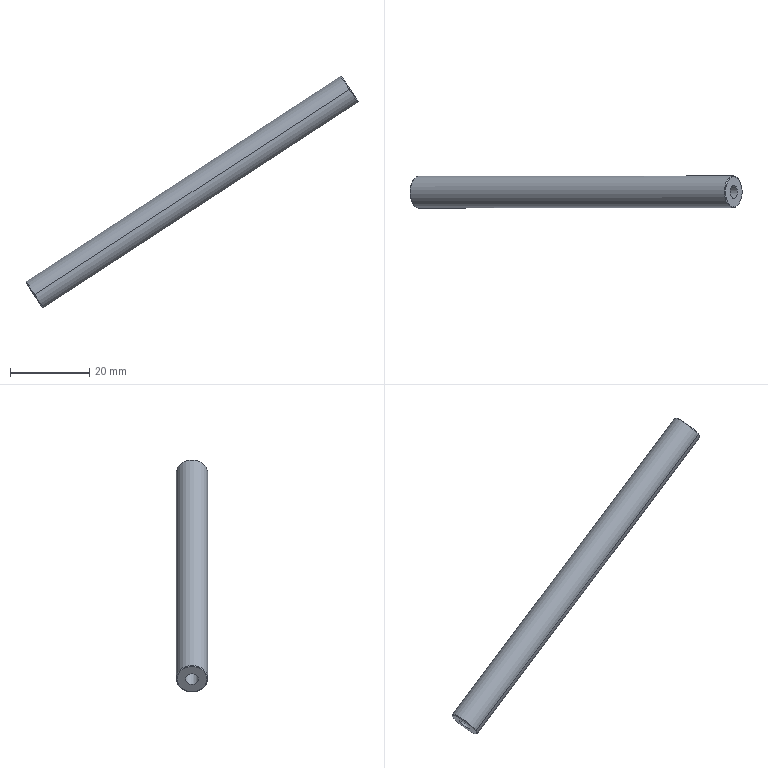Component | SolidWorks | NewSuctionCupGroup-1_GuideRod01-2 | 1 solid | 16 faces | box 83.68 x 8 x 58.45 mm | volume 4596 mm3 | cone 8 | cylinder 6 | plane 2 | commonest cylinder face diameters 3.3 x4 8 x2
build123d program:
from build123d import *

# Parameters (mm, degrees)
SKETCH1_R             = 4
BOSS_EXTRUDE1_DEPTH   = 95
CHAMFER1_SIZE         = 0.2
M4_TAPPED_HOLE1_D     = 3.3
M4_TAPPED_HOLE1_DEPTH = 10.1
M4_TAPPED_HOLE1_TIP   = 0.9914
M4_TAPPED_HOLE2_D     = 3.3
M4_TAPPED_HOLE2_DEPTH = 10.1
M4_TAPPED_HOLE2_TIP   = 0.9914


with BuildPart() as part:
    # Sketch1 → Boss-Extrude1 (new body)
    with BuildSketch(Plane.XY):
        Circle(SKETCH1_R)
    extrude(amount=BOSS_EXTRUDE1_DEPTH)

    # Chamfer1
    chamfer1_edges = [part.edges().sort_by_distance(p)[0] for p in [
        (-4, 0, 0),
        (-4, 0, 95),
    ]]
    chamfer(chamfer1_edges, length=CHAMFER1_SIZE)

    # M4 Tapped Hole1
    with Locations(Plane.XY.offset(95)):
        with Locations((0, 0)):
            Hole(M4_TAPPED_HOLE1_D / 2, depth=M4_TAPPED_HOLE1_DEPTH)
            with Locations((0, 0, -(M4_TAPPED_HOLE1_DEPTH + M4_TAPPED_HOLE1_TIP / 2))):  # 118° drill point
                Cone(0, M4_TAPPED_HOLE1_D / 2, M4_TAPPED_HOLE1_TIP, mode=Mode.SUBTRACT)

    # M4 Tapped Hole2
    with Locations(Plane(origin=(0, 0, 0), x_dir=(-1, 0, 0), z_dir=(0, 0, -1))):
        with Locations((0, 0)):
            Hole(M4_TAPPED_HOLE2_D / 2, depth=M4_TAPPED_HOLE2_DEPTH)
            with Locations((0, 0, -(M4_TAPPED_HOLE2_DEPTH + M4_TAPPED_HOLE2_TIP / 2))):  # 118° drill point
                Cone(0, M4_TAPPED_HOLE2_D / 2, M4_TAPPED_HOLE2_TIP, mode=Mode.SUBTRACT)


solid = part.part

# Placed as in the assembly
solid = solid.moved(Location((-73.051, -140.454, -18.564), (0, 56.835, 67.886)))
STEP:
#1=CARTESIAN_POINT('',(-0.07801,-5.595,1.098));
#2=VERTEX_POINT('',#1);
#3=CARTESIAN_POINT('',(-0.07801,-5.465,1.098));
#4=VERTEX_POINT('',#3);
#5=CARTESIAN_POINT('',(-0.07801,-5.53,1.098));
#6=DIRECTION('',(0.8371,-0.,0.5471));
#7=DIRECTION('',(0.,1.,0.));
#8=AXIS2_PLACEMENT_3D('',#5,#6,#7);
#9=CIRCLE('',#8,0.06496);
#10=EDGE_CURVE('',#2,#4,#9,.T.);
#11=ORIENTED_EDGE('',*,*,#10,.F.);
#12=CARTESIAN_POINT('',(0.2548,-5.595,1.315));
#13=VERTEX_POINT('',#12);
#14=CARTESIAN_POINT('',(0.2548,-5.595,1.315));
#15=DIRECTION('',(0.8371,-0.,0.5471));
#16=VECTOR('',#15,39.37);
#17=LINE('',#14,#16);
#18=EDGE_CURVE('',#2,#13,#17,.T.);
#19=ORIENTED_EDGE('',*,*,#18,.T.);
#20=CARTESIAN_POINT('',(0.2548,-5.465,1.315));
#21=VERTEX_POINT('',#20);
#22=CARTESIAN_POINT('',(0.2548,-5.53,1.315));
#23=DIRECTION('',(0.8371,-0.,0.5471));
#24=DIRECTION('',(0.,1.,0.));
#25=AXIS2_PLACEMENT_3D('',#22,#23,#24);
#26=CIRCLE('',#25,0.06496);
#27=EDGE_CURVE('',#13,#21,#26,.T.);
#28=ORIENTED_EDGE('',*,*,#27,.T.);
#29=CARTESIAN_POINT('',(0.2548,-5.465,1.315));
#30=DIRECTION('',(0.8371,-0.,0.5471));
#31=VECTOR('',#30,39.37);
#32=LINE('',#29,#31);
#33=EDGE_CURVE('',#4,#21,#32,.T.);
#34=ORIENTED_EDGE('',*,*,#33,.F.);
#35=EDGE_LOOP('',(#11,#19,#28,#34));
#36=FACE_OUTER_BOUND('',#35,.T.);
#37=CARTESIAN_POINT('',(0.2548,-5.53,1.315));
#38=DIRECTION('',(0.8371,-0.,0.5471));
#39=DIRECTION('',(0.,1.,0.));
#40=AXIS2_PLACEMENT_3D('',#37,#38,#39);
#41=CYLINDRICAL_SURFACE('',#40,0.06496);
#42=ADVANCED_FACE('',(#36),#41,.F.);
#43=CARTESIAN_POINT('',(-0.1107,-5.53,1.076));
#44=VERTEX_POINT('',#43);
#45=CARTESIAN_POINT('',(-0.07801,-5.465,1.098));
#46=DIRECTION('',(0.4311,0.8572,0.2818));
#47=VECTOR('',#46,39.37);
#48=LINE('',#45,#47);
#49=EDGE_CURVE('',#44,#4,#48,.T.);
#50=ORIENTED_EDGE('',*,*,#49,.F.);
#51=CARTESIAN_POINT('',(-0.07801,-5.595,1.098));
#52=DIRECTION('',(0.4311,-0.8572,0.2818));
#53=VECTOR('',#52,39.37);
#54=LINE('',#51,#53);
#55=EDGE_CURVE('',#44,#2,#54,.T.);
#56=ORIENTED_EDGE('',*,*,#55,.T.);
#57=ORIENTED_EDGE('',*,*,#10,.T.);
#58=EDGE_LOOP('',(#50,#56,#57));
#59=FACE_OUTER_BOUND('',#58,.T.);
#60=CARTESIAN_POINT('',(-0.07801,-5.53,1.098));
#61=DIRECTION('',(0.8371,-0.,0.5471));
#62=DIRECTION('',(0.,1.,0.));
#63=AXIS2_PLACEMENT_3D('',#60,#61,#62);
#64=CONICAL_SURFACE('',#63,0.06496,1.03);
#65=ADVANCED_FACE('',(#59),#64,.F.);
#66=CARTESIAN_POINT('',(-2.543,-5.465,-0.5133));
#67=VERTEX_POINT('',#66);
#68=CARTESIAN_POINT('',(-2.543,-5.595,-0.5133));
#69=VERTEX_POINT('',#68);
#70=CARTESIAN_POINT('',(-2.543,-5.53,-0.5133));
#71=DIRECTION('',(-0.8371,0.,-0.5471));
#72=DIRECTION('',(0.,-1.,0.));
#73=AXIS2_PLACEMENT_3D('',#70,#71,#72);
#74=CIRCLE('',#73,0.06496);
#75=EDGE_CURVE('',#67,#69,#74,.T.);
#76=ORIENTED_EDGE('',*,*,#75,.F.);
#77=CARTESIAN_POINT('',(-2.876,-5.465,-0.7309));
#78=VERTEX_POINT('',#77);
#79=CARTESIAN_POINT('',(-2.876,-5.465,-0.7309));
#80=DIRECTION('',(-0.8371,0.,-0.5471));
#81=VECTOR('',#80,39.37);
#82=LINE('',#79,#81);
#83=EDGE_CURVE('',#67,#78,#82,.T.);
#84=ORIENTED_EDGE('',*,*,#83,.T.);
#85=CARTESIAN_POINT('',(-2.876,-5.595,-0.7309));
#86=VERTEX_POINT('',#85);
#87=CARTESIAN_POINT('',(-2.876,-5.53,-0.7309));
#88=DIRECTION('',(-0.8371,0.,-0.5471));
#89=DIRECTION('',(0.,-1.,0.));
#90=AXIS2_PLACEMENT_3D('',#87,#88,#89);
#91=CIRCLE('',#90,0.06496);
#92=EDGE_CURVE('',#78,#86,#91,.T.);
#93=ORIENTED_EDGE('',*,*,#92,.T.);
#94=CARTESIAN_POINT('',(-2.876,-5.595,-0.7309));
#95=DIRECTION('',(-0.8371,0.,-0.5471));
#96=VECTOR('',#95,39.37);
#97=LINE('',#94,#96);
#98=EDGE_CURVE('',#69,#86,#97,.T.);
#99=ORIENTED_EDGE('',*,*,#98,.F.);
#100=EDGE_LOOP('',(#76,#84,#93,#99));
#101=FACE_OUTER_BOUND('',#100,.T.);
#102=CARTESIAN_POINT('',(-2.876,-5.53,-0.7309));
#103=DIRECTION('',(-0.8371,0.,-0.5471));
#104=DIRECTION('',(0.,-1.,0.));
#105=AXIS2_PLACEMENT_3D('',#102,#103,#104);
#106=CYLINDRICAL_SURFACE('',#105,0.06496);
#107=ADVANCED_FACE('',(#101),#106,.F.);
#108=CARTESIAN_POINT('',(-2.51,-5.53,-0.492));
#109=VERTEX_POINT('',#108);
#110=CARTESIAN_POINT('',(-2.543,-5.595,-0.5133));
#111=DIRECTION('',(-0.4311,-0.8572,-0.2818));
#112=VECTOR('',#111,39.37);
#113=LINE('',#110,#112);
#114=EDGE_CURVE('',#109,#69,#113,.T.);
#115=ORIENTED_EDGE('',*,*,#114,.F.);
#116=CARTESIAN_POINT('',(-2.543,-5.465,-0.5133));
#117=DIRECTION('',(-0.4311,0.8572,-0.2818));
#118=VECTOR('',#117,39.37);
#119=LINE('',#116,#118);
#120=EDGE_CURVE('',#109,#67,#119,.T.);
#121=ORIENTED_EDGE('',*,*,#120,.T.);
#122=ORIENTED_EDGE('',*,*,#75,.T.);
#123=EDGE_LOOP('',(#115,#121,#122));
#124=FACE_OUTER_BOUND('',#123,.T.);
#125=CARTESIAN_POINT('',(-2.543,-5.53,-0.5133));
#126=DIRECTION('',(-0.8371,0.,-0.5471));
#127=DIRECTION('',(0.,-1.,0.));
#128=AXIS2_PLACEMENT_3D('',#125,#126,#127);
#129=CONICAL_SURFACE('',#128,0.06496,1.03);
#130=ADVANCED_FACE('',(#124),#129,.F.);
#131=CARTESIAN_POINT('',(-2.876,-5.679,-0.7309));
#132=VERTEX_POINT('',#131);
#133=CARTESIAN_POINT('',(-2.876,-5.38,-0.7309));
#134=VERTEX_POINT('',#133);
#135=CARTESIAN_POINT('',(-2.876,-5.53,-0.7309));
#136=DIRECTION('',(-0.8371,0.,-0.5471));
#137=DIRECTION('',(0.,-1.,0.));
#138=AXIS2_PLACEMENT_3D('',#135,#136,#137);
#139=CIRCLE('',#138,0.1496);
#140=EDGE_CURVE('',#132,#134,#139,.T.);
#141=ORIENTED_EDGE('',*,*,#140,.F.);
#142=CARTESIAN_POINT('',(-2.869,-5.687,-0.7266));
#143=VERTEX_POINT('',#142);
#144=CARTESIAN_POINT('',(-2.876,-5.679,-0.7309));
#145=DIRECTION('',(0.5919,-0.7071,0.3868));
#146=VECTOR('',#145,39.37);
#147=LINE('',#144,#146);
#148=EDGE_CURVE('',#132,#143,#147,.T.);
#149=ORIENTED_EDGE('',*,*,#148,.T.);
#150=CARTESIAN_POINT('',(-2.869,-5.372,-0.7266));
#151=VERTEX_POINT('',#150);
#152=CARTESIAN_POINT('',(-2.869,-5.53,-0.7266));
#153=DIRECTION('',(0.8371,-0.,0.5471));
#154=DIRECTION('',(0.,-1.,-0.));
#155=AXIS2_PLACEMENT_3D('',#152,#153,#154);
#156=CIRCLE('',#155,0.1575);
#157=EDGE_CURVE('',#151,#143,#156,.T.);
#158=ORIENTED_EDGE('',*,*,#157,.F.);
#159=CARTESIAN_POINT('',(-2.876,-5.38,-0.7309));
#160=DIRECTION('',(0.5919,0.7071,0.3868));
#161=VECTOR('',#160,39.37);
#162=LINE('',#159,#161);
#163=EDGE_CURVE('',#134,#151,#162,.T.);
#164=ORIENTED_EDGE('',*,*,#163,.F.);
#165=EDGE_LOOP('',(#141,#149,#158,#164));
#166=FACE_OUTER_BOUND('',#165,.T.);
#167=CARTESIAN_POINT('',(-2.876,-5.53,-0.7309));
#168=DIRECTION('',(0.8371,-0.,0.5471));
#169=DIRECTION('',(0.,1.,-0.));
#170=AXIS2_PLACEMENT_3D('',#167,#168,#169);
#171=CONICAL_SURFACE('',#170,0.1496,0.7854);
#172=ADVANCED_FACE('',(#166),#171,.T.);
#173=CARTESIAN_POINT('',(0.2548,-5.38,1.315));
#174=VERTEX_POINT('',#173);
#175=CARTESIAN_POINT('',(0.2548,-5.679,1.315));
#176=VERTEX_POINT('',#175);
#177=CARTESIAN_POINT('',(0.2548,-5.53,1.315));
#178=DIRECTION('',(0.8371,-0.,0.5471));
#179=DIRECTION('',(-0.,-1.,0.));
#180=AXIS2_PLACEMENT_3D('',#177,#178,#179);
#181=CIRCLE('',#180,0.1496);
#182=EDGE_CURVE('',#174,#176,#181,.T.);
#183=ORIENTED_EDGE('',*,*,#182,.F.);
#184=CARTESIAN_POINT('',(0.2483,-5.372,1.311));
#185=VERTEX_POINT('',#184);
#186=CARTESIAN_POINT('',(0.2483,-5.372,1.311));
#187=DIRECTION('',(-0.5919,0.7071,-0.3868));
#188=VECTOR('',#187,39.37);
#189=LINE('',#186,#188);
#190=EDGE_CURVE('',#174,#185,#189,.T.);
#191=ORIENTED_EDGE('',*,*,#190,.T.);
#192=CARTESIAN_POINT('',(0.2483,-5.687,1.311));
#193=VERTEX_POINT('',#192);
#194=CARTESIAN_POINT('',(0.2483,-5.53,1.311));
#195=DIRECTION('',(-0.8371,0.,-0.5471));
#196=DIRECTION('',(-0.,-1.,0.));
#197=AXIS2_PLACEMENT_3D('',#194,#195,#196);
#198=CIRCLE('',#197,0.1575);
#199=EDGE_CURVE('',#193,#185,#198,.T.);
#200=ORIENTED_EDGE('',*,*,#199,.F.);
#201=CARTESIAN_POINT('',(0.2483,-5.687,1.311));
#202=DIRECTION('',(-0.5919,-0.7071,-0.3868));
#203=VECTOR('',#202,39.37);
#204=LINE('',#201,#203);
#205=EDGE_CURVE('',#176,#193,#204,.T.);
#206=ORIENTED_EDGE('',*,*,#205,.F.);
#207=EDGE_LOOP('',(#183,#191,#200,#206));
#208=FACE_OUTER_BOUND('',#207,.T.);
#209=CARTESIAN_POINT('',(0.2483,-5.53,1.311));
#210=DIRECTION('',(-0.8371,0.,-0.5471));
#211=DIRECTION('',(-0.,-1.,0.));
#212=AXIS2_PLACEMENT_3D('',#209,#210,#211);
#213=CONICAL_SURFACE('',#212,0.1575,0.7854);
#214=ADVANCED_FACE('',(#208),#213,.T.);
#215=ORIENTED_EDGE('',*,*,#157,.T.);
#216=CARTESIAN_POINT('',(-2.876,-5.687,-0.7309));
#217=DIRECTION('',(0.8371,-0.,0.5471));
#218=VECTOR('',#217,39.37);
#219=LINE('',#216,#218);
#220=EDGE_CURVE('',#143,#193,#219,.T.);
#221=ORIENTED_EDGE('',*,*,#220,.T.);
#222=ORIENTED_EDGE('',*,*,#199,.T.);
#223=CARTESIAN_POINT('',(-2.876,-5.372,-0.7309));
#224=DIRECTION('',(0.8371,-0.,0.5471));
#225=VECTOR('',#224,39.37);
#226=LINE('',#223,#225);
#227=EDGE_CURVE('',#151,#185,#226,.T.);
#228=ORIENTED_EDGE('',*,*,#227,.F.);
#229=EDGE_LOOP('',(#215,#221,#222,#228));
#230=FACE_OUTER_BOUND('',#229,.T.);
#231=CARTESIAN_POINT('',(-2.876,-5.53,-0.7309));
#232=DIRECTION('',(0.8371,-0.,0.5471));
#233=DIRECTION('',(0.,1.,-0.));
#234=AXIS2_PLACEMENT_3D('',#231,#232,#233);
#235=CYLINDRICAL_SURFACE('',#234,0.1575);
#236=ADVANCED_FACE('',(#230),#235,.T.);
#237=ORIENTED_EDGE('',*,*,#220,.F.);
#238=CARTESIAN_POINT('',(-2.869,-5.53,-0.7266));
#239=DIRECTION('',(0.8371,-0.,0.5471));
#240=DIRECTION('',(-0.,-1.,0.));
#241=AXIS2_PLACEMENT_3D('',#238,#239,#240);
#242=CIRCLE('',#241,0.1575);
#243=EDGE_CURVE('',#143,#151,#242,.T.);
#244=ORIENTED_EDGE('',*,*,#243,.T.);
#245=ORIENTED_EDGE('',*,*,#227,.T.);
#246=CARTESIAN_POINT('',(0.2483,-5.53,1.311));
#247=DIRECTION('',(-0.8371,0.,-0.5471));
#248=DIRECTION('',(-0.,-1.,0.));
#249=AXIS2_PLACEMENT_3D('',#246,#247,#248);
#250=CIRCLE('',#249,0.1575);
#251=EDGE_CURVE('',#185,#193,#250,.T.);
#252=ORIENTED_EDGE('',*,*,#251,.T.);
#253=EDGE_LOOP('',(#237,#244,#245,#252));
#254=FACE_OUTER_BOUND('',#253,.T.);
#255=CARTESIAN_POINT('',(-2.876,-5.53,-0.7309));
#256=DIRECTION('',(0.8371,-0.,0.5471));
#257=DIRECTION('',(0.,1.,-0.));
#258=AXIS2_PLACEMENT_3D('',#255,#256,#257);
#259=CYLINDRICAL_SURFACE('',#258,0.1575);
#260=ADVANCED_FACE('',(#254),#259,.T.);
#261=CARTESIAN_POINT('',(-2.876,-5.53,-0.7309));
#262=DIRECTION('',(-0.8371,0.,-0.5471));
#263=DIRECTION('',(0.,-1.,0.));
#264=AXIS2_PLACEMENT_3D('',#261,#262,#263);
#265=CIRCLE('',#264,0.06496);
#266=EDGE_CURVE('',#86,#78,#265,.T.);
#267=ORIENTED_EDGE('',*,*,#266,.F.);
#268=ORIENTED_EDGE('',*,*,#92,.F.);
#269=EDGE_LOOP('',(#267,#268));
#270=FACE_BOUND('',#269,.T.);
#271=CARTESIAN_POINT('',(-2.876,-5.53,-0.7309));
#272=DIRECTION('',(-0.8371,0.,-0.5471));
#273=DIRECTION('',(0.,-1.,0.));
#274=AXIS2_PLACEMENT_3D('',#271,#272,#273);
#275=CIRCLE('',#274,0.1496);
#276=EDGE_CURVE('',#134,#132,#275,.T.);
#277=ORIENTED_EDGE('',*,*,#276,.T.);
#278=ORIENTED_EDGE('',*,*,#140,.T.);
#279=EDGE_LOOP('',(#277,#278));
#280=FACE_OUTER_BOUND('',#279,.T.);
#281=CARTESIAN_POINT('',(-2.876,-5.53,-0.7309));
#282=DIRECTION('',(-0.8371,0.,-0.5471));
#283=DIRECTION('',(-0.,-1.,0.));
#284=AXIS2_PLACEMENT_3D('',#281,#282,#283);
#285=PLANE('',#284);
#286=ADVANCED_FACE('',(#270,#280),#285,.T.);
#287=CARTESIAN_POINT('',(0.2548,-5.53,1.315));
#288=DIRECTION('',(0.8371,-0.,0.5471));
#289=DIRECTION('',(0.,1.,0.));
#290=AXIS2_PLACEMENT_3D('',#287,#288,#289);
#291=CIRCLE('',#290,0.06496);
#292=EDGE_CURVE('',#21,#13,#291,.T.);
#293=ORIENTED_EDGE('',*,*,#292,.F.);
#294=ORIENTED_EDGE('',*,*,#27,.F.);
#295=EDGE_LOOP('',(#293,#294));
#296=FACE_BOUND('',#295,.T.);
#297=CARTESIAN_POINT('',(0.2548,-5.53,1.315));
#298=DIRECTION('',(0.8371,-0.,0.5471));
#299=DIRECTION('',(-0.,-1.,0.));
#300=AXIS2_PLACEMENT_3D('',#297,#298,#299);
#301=CIRCLE('',#300,0.1496);
#302=EDGE_CURVE('',#176,#174,#301,.T.);
#303=ORIENTED_EDGE('',*,*,#302,.T.);
#304=ORIENTED_EDGE('',*,*,#182,.T.);
#305=EDGE_LOOP('',(#303,#304));
#306=FACE_OUTER_BOUND('',#305,.T.);
#307=CARTESIAN_POINT('',(0.2548,-5.53,1.315));
#308=DIRECTION('',(-0.8371,0.,-0.5471));
#309=DIRECTION('',(-0.,-1.,0.));
#310=AXIS2_PLACEMENT_3D('',#307,#308,#309);
#311=PLANE('',#310);
#312=ADVANCED_FACE('',(#296,#306),#311,.F.);
#313=ORIENTED_EDGE('',*,*,#190,.F.);
#314=ORIENTED_EDGE('',*,*,#302,.F.);
#315=ORIENTED_EDGE('',*,*,#205,.T.);
#316=ORIENTED_EDGE('',*,*,#251,.F.);
#317=EDGE_LOOP('',(#313,#314,#315,#316));
#318=FACE_OUTER_BOUND('',#317,.T.);
#319=CARTESIAN_POINT('',(0.2483,-5.53,1.311));
#320=DIRECTION('',(-0.8371,0.,-0.5471));
#321=DIRECTION('',(-0.,-1.,0.));
#322=AXIS2_PLACEMENT_3D('',#319,#320,#321);
#323=CONICAL_SURFACE('',#322,0.1575,0.7854);
#324=ADVANCED_FACE('',(#318),#323,.T.);
#325=ORIENTED_EDGE('',*,*,#148,.F.);
#326=ORIENTED_EDGE('',*,*,#276,.F.);
#327=ORIENTED_EDGE('',*,*,#163,.T.);
#328=ORIENTED_EDGE('',*,*,#243,.F.);
#329=EDGE_LOOP('',(#325,#326,#327,#328));
#330=FACE_OUTER_BOUND('',#329,.T.);
#331=CARTESIAN_POINT('',(-2.876,-5.53,-0.7309));
#332=DIRECTION('',(0.8371,-0.,0.5471));
#333=DIRECTION('',(0.,1.,-0.));
#334=AXIS2_PLACEMENT_3D('',#331,#332,#333);
#335=CONICAL_SURFACE('',#334,0.1496,0.7854);
#336=ADVANCED_FACE('',(#330),#335,.T.);
#337=ORIENTED_EDGE('',*,*,#120,.F.);
#338=ORIENTED_EDGE('',*,*,#114,.T.);
#339=CARTESIAN_POINT('',(-2.543,-5.53,-0.5133));
#340=DIRECTION('',(-0.8371,0.,-0.5471));
#341=DIRECTION('',(0.,-1.,0.));
#342=AXIS2_PLACEMENT_3D('',#339,#340,#341);
#343=CIRCLE('',#342,0.06496);
#344=EDGE_CURVE('',#69,#67,#343,.T.);
#345=ORIENTED_EDGE('',*,*,#344,.T.);
#346=EDGE_LOOP('',(#337,#338,#345));
#347=FACE_OUTER_BOUND('',#346,.T.);
#348=CARTESIAN_POINT('',(-2.543,-5.53,-0.5133));
#349=DIRECTION('',(-0.8371,0.,-0.5471));
#350=DIRECTION('',(0.,-1.,0.));
#351=AXIS2_PLACEMENT_3D('',#348,#349,#350);
#352=CONICAL_SURFACE('',#351,0.06496,1.03);
#353=ADVANCED_FACE('',(#347),#352,.F.);
#354=ORIENTED_EDGE('',*,*,#83,.F.);
#355=ORIENTED_EDGE('',*,*,#344,.F.);
#356=ORIENTED_EDGE('',*,*,#98,.T.);
#357=ORIENTED_EDGE('',*,*,#266,.T.);
#358=EDGE_LOOP('',(#354,#355,#356,#357));
#359=FACE_OUTER_BOUND('',#358,.T.);
#360=CARTESIAN_POINT('',(-2.876,-5.53,-0.7309));
#361=DIRECTION('',(-0.8371,0.,-0.5471));
#362=DIRECTION('',(0.,-1.,0.));
#363=AXIS2_PLACEMENT_3D('',#360,#361,#362);
#364=CYLINDRICAL_SURFACE('',#363,0.06496);
#365=ADVANCED_FACE('',(#359),#364,.F.);
#366=ORIENTED_EDGE('',*,*,#55,.F.);
#367=ORIENTED_EDGE('',*,*,#49,.T.);
#368=CARTESIAN_POINT('',(-0.07801,-5.53,1.098));
#369=DIRECTION('',(0.8371,-0.,0.5471));
#370=DIRECTION('',(0.,1.,0.));
#371=AXIS2_PLACEMENT_3D('',#368,#369,#370);
#372=CIRCLE('',#371,0.06496);
#373=EDGE_CURVE('',#4,#2,#372,.T.);
#374=ORIENTED_EDGE('',*,*,#373,.T.);
#375=EDGE_LOOP('',(#366,#367,#374));
#376=FACE_OUTER_BOUND('',#375,.T.);
#377=CARTESIAN_POINT('',(-0.07801,-5.53,1.098));
#378=DIRECTION('',(0.8371,-0.,0.5471));
#379=DIRECTION('',(0.,1.,0.));
#380=AXIS2_PLACEMENT_3D('',#377,#378,#379);
#381=CONICAL_SURFACE('',#380,0.06496,1.03);
#382=ADVANCED_FACE('',(#376),#381,.F.);
#383=ORIENTED_EDGE('',*,*,#18,.F.);
#384=ORIENTED_EDGE('',*,*,#373,.F.);
#385=ORIENTED_EDGE('',*,*,#33,.T.);
#386=ORIENTED_EDGE('',*,*,#292,.T.);
#387=EDGE_LOOP('',(#383,#384,#385,#386));
#388=FACE_OUTER_BOUND('',#387,.T.);
#389=CARTESIAN_POINT('',(0.2548,-5.53,1.315));
#390=DIRECTION('',(0.8371,-0.,0.5471));
#391=DIRECTION('',(0.,1.,0.));
#392=AXIS2_PLACEMENT_3D('',#389,#390,#391);
#393=CYLINDRICAL_SURFACE('',#392,0.06496);
#394=ADVANCED_FACE('',(#388),#393,.F.);
#395=CLOSED_SHELL('',(#42,#65,#107,#130,#172,#214,#236,#260,#286,#312,#324,#336,#353,#365,#382,#394));
#396=MANIFOLD_SOLID_BREP('',#395);
#397=CARTESIAN_POINT('',(0.,0.,0.));
#398=DIRECTION('',(0.,0.,1.));
#399=DIRECTION('',(1.,0.,0.));
#400=AXIS2_PLACEMENT_3D('',#397,#398,#399);
#401=(LENGTH_UNIT()NAMED_UNIT(*)SI_UNIT($,.METRE.));
#402=LENGTH_MEASURE_WITH_UNIT(LENGTH_MEASURE(0.0254),#401);
#403=DIMENSIONAL_EXPONENTS(1.,0.,0.,0.,0.,0.,0.);
#404=(CONVERSION_BASED_UNIT('',#402)LENGTH_UNIT()NAMED_UNIT(#403));
#405=UNCERTAINTY_MEASURE_WITH_UNIT(LENGTH_MEASURE(0.00001),#404,'','');
#406=(NAMED_UNIT(*)PLANE_ANGLE_UNIT()SI_UNIT($,.RADIAN.));
#407=(NAMED_UNIT(*)SI_UNIT($,.STERADIAN.)SOLID_ANGLE_UNIT());
#408=(GEOMETRIC_REPRESENTATION_CONTEXT(3)GLOBAL_UNCERTAINTY_ASSIGNED_CONTEXT((#405))GLOBAL_UNIT_ASSIGNED_CONTEXT((#404,#406,#407))REPRESENTATION_CONTEXT('',''));
#409=ADVANCED_BREP_SHAPE_REPRESENTATION('',(#396,#400),#408);
#410=COLOUR_RGB('',0.7922,0.8196,0.9333);
#411=FILL_AREA_STYLE_COLOUR('',#410);
#412=FILL_AREA_STYLE('',(#411));
#413=SURFACE_STYLE_FILL_AREA(#412);
#414=SURFACE_SIDE_STYLE('',(#413));
#415=SURFACE_STYLE_USAGE(.BOTH.,#414);
#416=PRESENTATION_STYLE_ASSIGNMENT((#415));
#417=STYLED_ITEM('',(#416),#396);
#418=(LENGTH_UNIT()NAMED_UNIT(*)SI_UNIT($,.METRE.));
#419=LENGTH_MEASURE_WITH_UNIT(LENGTH_MEASURE(0.0254),#418);
#420=DIMENSIONAL_EXPONENTS(1.,0.,0.,0.,0.,0.,0.);
#421=(CONVERSION_BASED_UNIT('',#419)LENGTH_UNIT()NAMED_UNIT(#420));
#422=UNCERTAINTY_MEASURE_WITH_UNIT(LENGTH_MEASURE(0.00001),#421,'','');
#423=(NAMED_UNIT(*)PLANE_ANGLE_UNIT()SI_UNIT($,.RADIAN.));
#424=(NAMED_UNIT(*)SI_UNIT($,.STERADIAN.)SOLID_ANGLE_UNIT());
#425=(GEOMETRIC_REPRESENTATION_CONTEXT(3)GLOBAL_UNCERTAINTY_ASSIGNED_CONTEXT((#422))GLOBAL_UNIT_ASSIGNED_CONTEXT((#421,#423,#424))REPRESENTATION_CONTEXT('',''));
#426=MECHANICAL_DESIGN_GEOMETRIC_PRESENTATION_REPRESENTATION('',(#417),#425);
#427=PRESENTATION_LAYER_ASSIGNMENT('','',(#417));